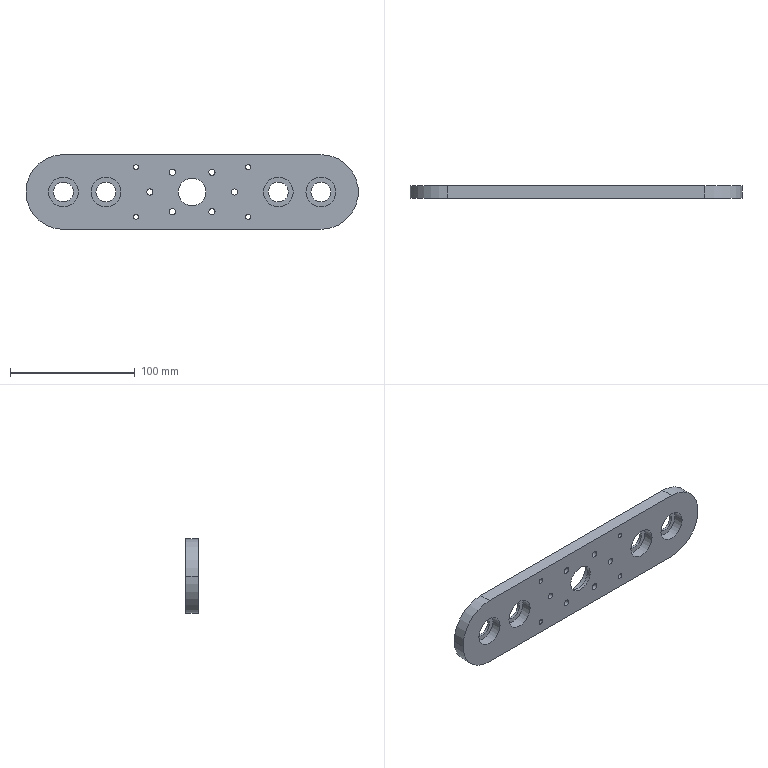Component | SolidWorks | UpperBracket-2 | 1 solid | 76 faces | volume 125796 mm3 | cylinder 59 | plane 17 | commonest cylinder face diameters 10 x16 5 x12 24 x8 16 x8 4 x8 60 x3 32 x2 22 x2 | material 6061-T6 (SS)